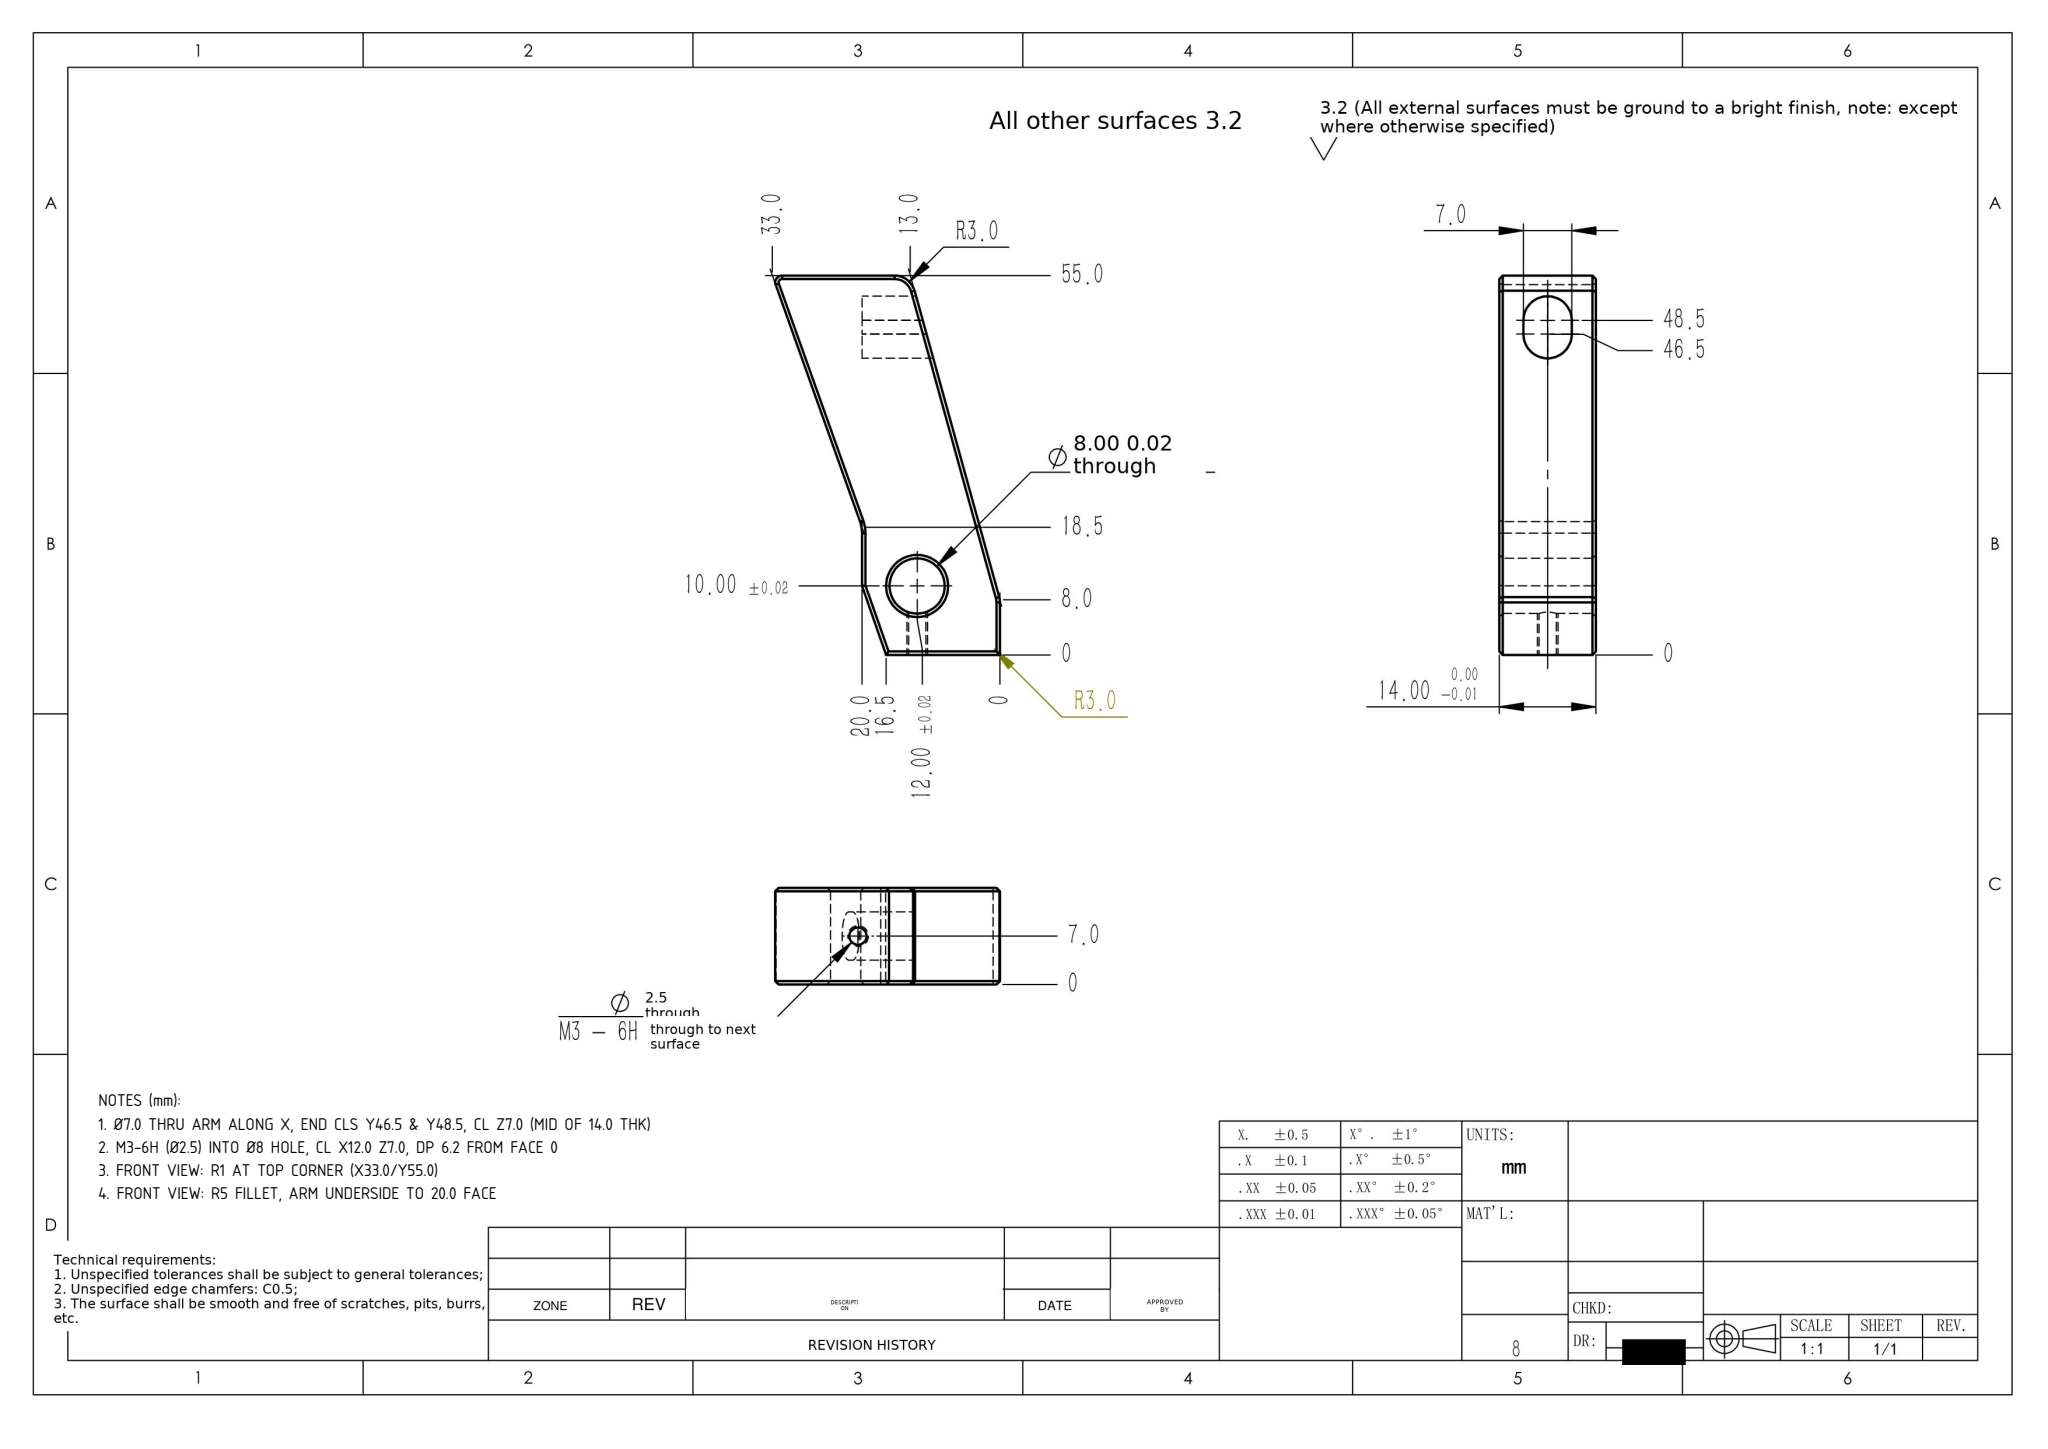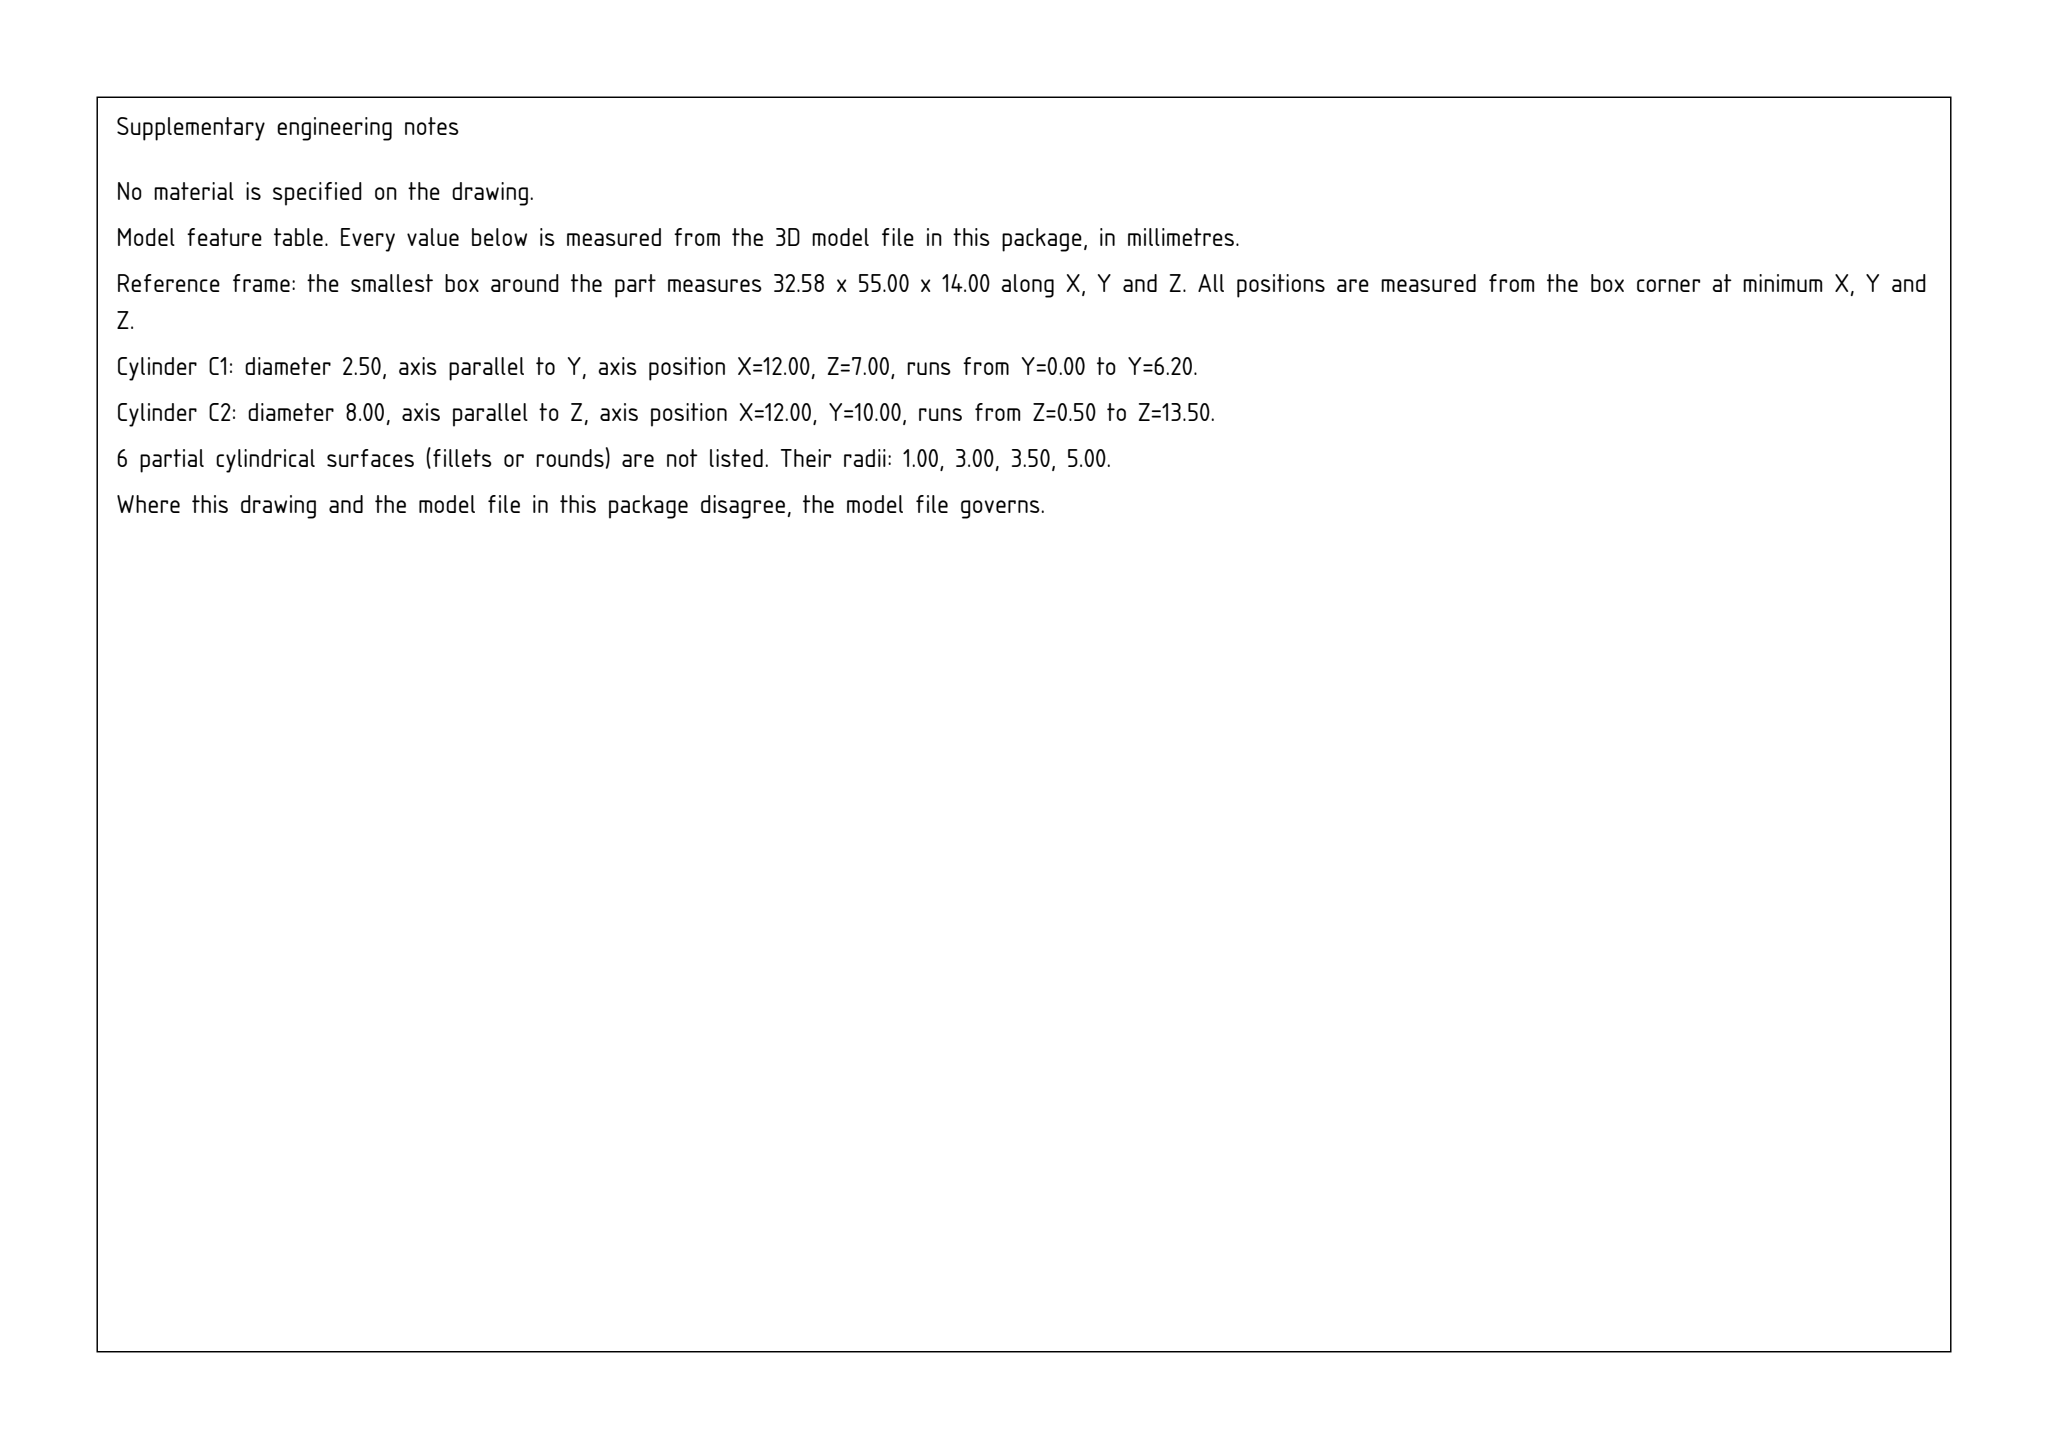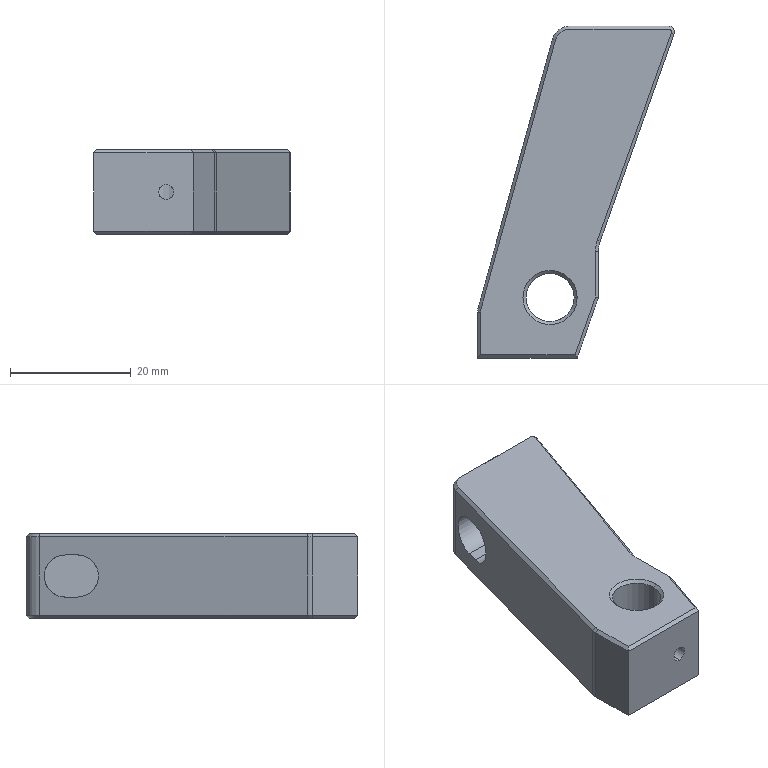Part | SolidWorks | mm | 1 solid | 49 faces | box 32.58 x 55 x 14 mm | volume 12926 mm3 | plane 26 | cone 13 | cylinder 10 | commonest cylinder face diameters 2.5 x2 8 x2 7 x2 6 x2 10 x1 2 x1
Drawing notes:
Ø7.0 THRU ARM ALONG X, END CLS Y46.5 & Y48.5, CL Z7.0 (MID OF 14.0 THK) | from the solid: cyls dia 7.0 axis x at y=46.5 (len 10.32) and y=48.5 (len 8.8), both z=7.0; thk 14.0
M3-6H (Ø2.5) INTO Ø8 HOLE, CL X12.0 Z7.0, DP 6.2 FROM FACE 0 | from the solid: cyl dia 2.5 axis y at x=12.0, z=7.0, length 6.2 (2 faces); Ø8 thru hole axis z at x=12.0
FRONT VIEW: R1 AT TOP CORNER (X33.0/Y55.0) | from the solid: cylinder dia 2.0, axis z, at x=31.58 y=54.0, len 13.0 -> R1 tangent at 33.0/55.0 corner
FRONT VIEW: R5 FILLET, ARM UNDERSIDE TO 20.0 FACE | from the solid: cylinder dia 10.0, axis z, at x=25.0 y=17.64, len 13.0 -> R5 tangent to plane x=20.0
build123d program:
from build123d import *

# Parameters (mm, degrees)
BOSS_EXTRUDE1_DEPTH    = 14
SKETCH2_R              = 4
CUT_EXTRUDE1_DEPTH     = 66.651
CUT_EXTRUDE2_DEPTH     = 20
M3_TAPPED_HOLE1_REACH  = 67.651
M3_TAPPED_HOLE1_BORE_R = 1.25
FILLET1_R              = 3
FILLET2_R              = 5
CHAMFER1_SIZE          = 3.5
CHAMFER1_SIZE2         = 10
FILLET3_R              = 1
CHAMFER2_SIZE          = 0.5


with BuildPart() as part:
    # Sketch1 → Boss-Extrude1 (new body)
    with BuildSketch(Plane.XY):
        Polygon((13, 55), (33, 55), (20, 18.5), (20, 0), (0, 0), (0, 8), align=None)
    extrude(amount=BOSS_EXTRUDE1_DEPTH)

    # Sketch2 → Cut-Extrude1 (cut, through all)
    with BuildSketch(Plane.XY.offset(14)):
        with Locations((12, 10)):
            Circle(SKETCH2_R)
    extrude(amount=-CUT_EXTRUDE1_DEPTH, mode=Mode.SUBTRACT)

    # Sketch4 → Cut-Extrude2 (cut)
    with BuildSketch(Plane(origin=(0, 15.621, 0), x_dir=(0, 0, 1), z_dir=(1, 0, 0))):
        with BuildLine():
            Line((3.5, -32.879), (3.5, -30.879))
            ThreePointArc((3.5, -30.879), (7, -27.379), (10.5, -30.879))
            Line((10.5, -30.879), (10.5, -32.879))
            ThreePointArc((10.5, -32.879), (7, -36.379), (3.5, -32.879))
        make_face()
    extrude(amount=CUT_EXTRUDE2_DEPTH, mode=Mode.SUBTRACT)

    # M3 Tapped Hole1 bore → M3 Tapped Hole1 (cut, up to next)
    with BuildSketch(Plane(origin=(0, 0, 0), x_dir=(-1, 0, 0), z_dir=(0, -1, 0)), mode=Mode.PRIVATE) as m3_tapped_hole1_sk1:
        with Locations((-12, -7)):
            Circle(M3_TAPPED_HOLE1_BORE_R)
    m3_tapped_hole1_tool1 = extrude(m3_tapped_hole1_sk1.sketch, amount=-M3_TAPPED_HOLE1_REACH, mode=Mode.PRIVATE) & part.part
    add(m3_tapped_hole1_tool1.solids().sort_by_distance((12, 0, 7))[0], mode=Mode.SUBTRACT)

    # Fillet1
    fillet1_edges = [part.edges().sort_by_distance(p)[0] for p in [
        (0, 8, 7),
        (13, 55, 7),
    ]]
    fillet(fillet1_edges, radius=FILLET1_R)

    # Fillet2
    fillet2_edges = [part.edges().sort_by_distance(p)[0] for p in [
        (20, 18.5, 7),
    ]]
    fillet(fillet2_edges, radius=FILLET2_R)

    # Chamfer1
    chamfer1_edges = [part.edges().sort_by_distance(p)[0] for p in [
        (20, 0, 7),
    ]]
    chamfer1_side = [part.faces().sort_by_distance(p)[0] for p in [
        (9.964, 0, 7),
    ]]
    chamfer(chamfer1_edges, length=CHAMFER1_SIZE, length2=CHAMFER1_SIZE2, reference=chamfer1_side[0])

    # Fillet3
    fillet3_edges = [part.edges().sort_by_distance(p)[0] for p in [
        (33, 55, 7),
    ]]
    fillet(fillet3_edges, radius=FILLET3_R)

    # Chamfer2
    chamfer2_edges = [part.edges().sort_by_distance(p)[0] for p in [
        (8, 10, 0),
        (8, 10, 14),
        (8.25, 0, 14),
        (6.25, 30.596, 0),
        (6.25, 30.596, 14),
        (0, 3.796, 0),
        (0.02727, 7.996, 0),
        (13.466, 54.387, 0),
        (0, 3.796, 14),
        (0.02727, 7.996, 14),
        (13.466, 54.387, 14),
        (26.407, 36.489, 0),
        (26.407, 36.489, 14),
        (20.073, 18.487, 0),
        (20.073, 18.487, 14),
        (20, 13.818, 0),
        (20, 13.818, 14),
        (18.25, 5, 0),
        (18.25, 5, 14),
        (23.433, 55, 0),
        (23.433, 55, 14),
        (32.399, 54.576, 0),
        (32.399, 54.576, 14),
        (8.25, 0, 0),
    ]]
    chamfer(chamfer2_edges, length=CHAMFER2_SIZE)


solid = part.part